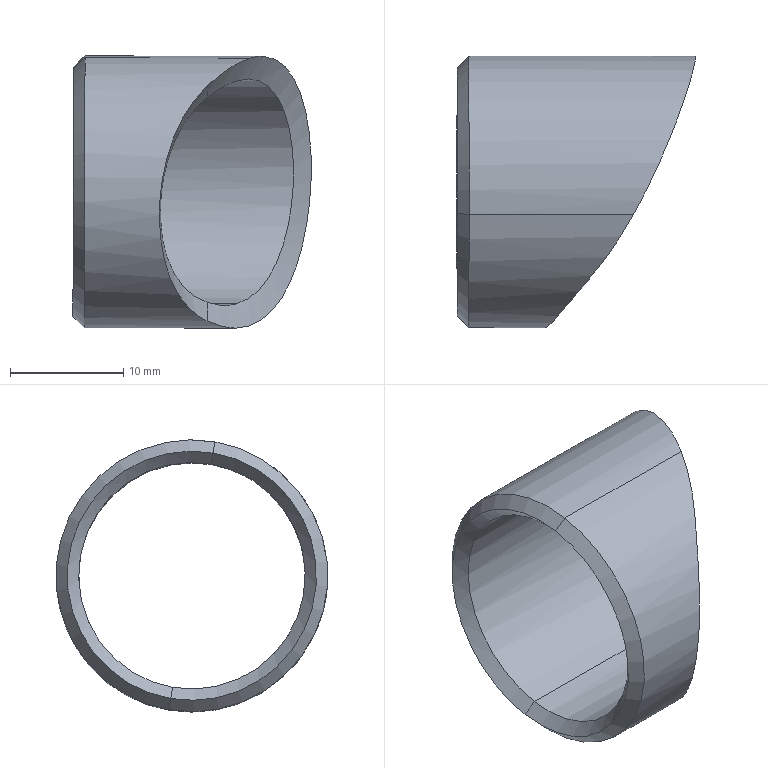Component | SolidWorks | Eyepiece-1 | 1 solid | 10 faces | box 21.04 x 24 x 24.04 mm | volume 1918 mm3 | cone 5 | cylinder 4 | torus 1 | commonest cylinder face diameters 20 x2 24 x2